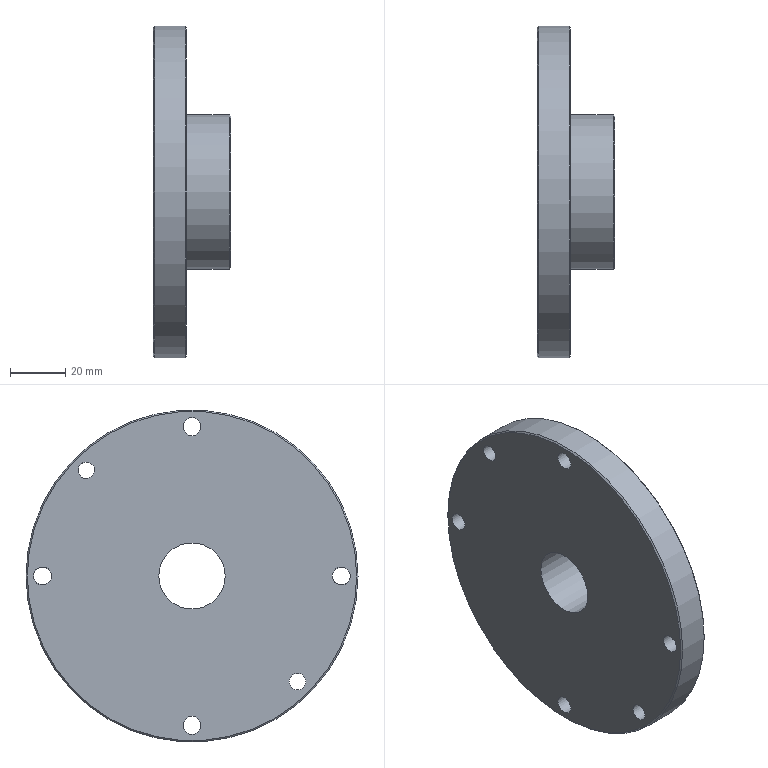Component | NX | END_CAP | 1 solid | 15 faces | volume 160071 mm3 | cylinder 9 | plane 3 | cone 3 | commonest cylinder face diameters 6.5 x4 6 x2 120 x1 56 x1 24 x1